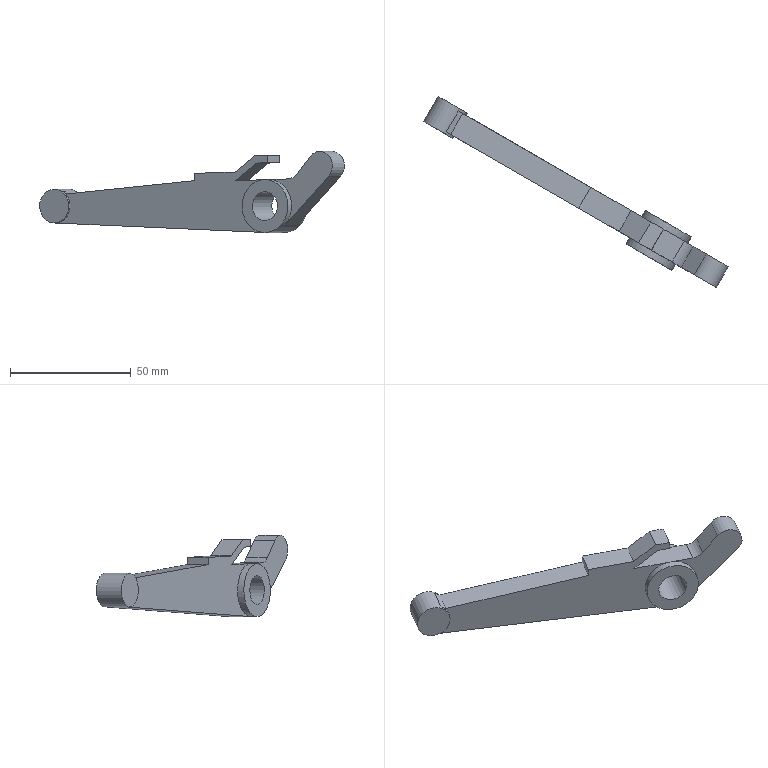Component | NX | TOGGLE_LEVER | 1 solid | 26 faces | volume 25756 mm3 | plane 21 | cylinder 5 | commonest cylinder face diameters 12 x3 14 x1 22 x1